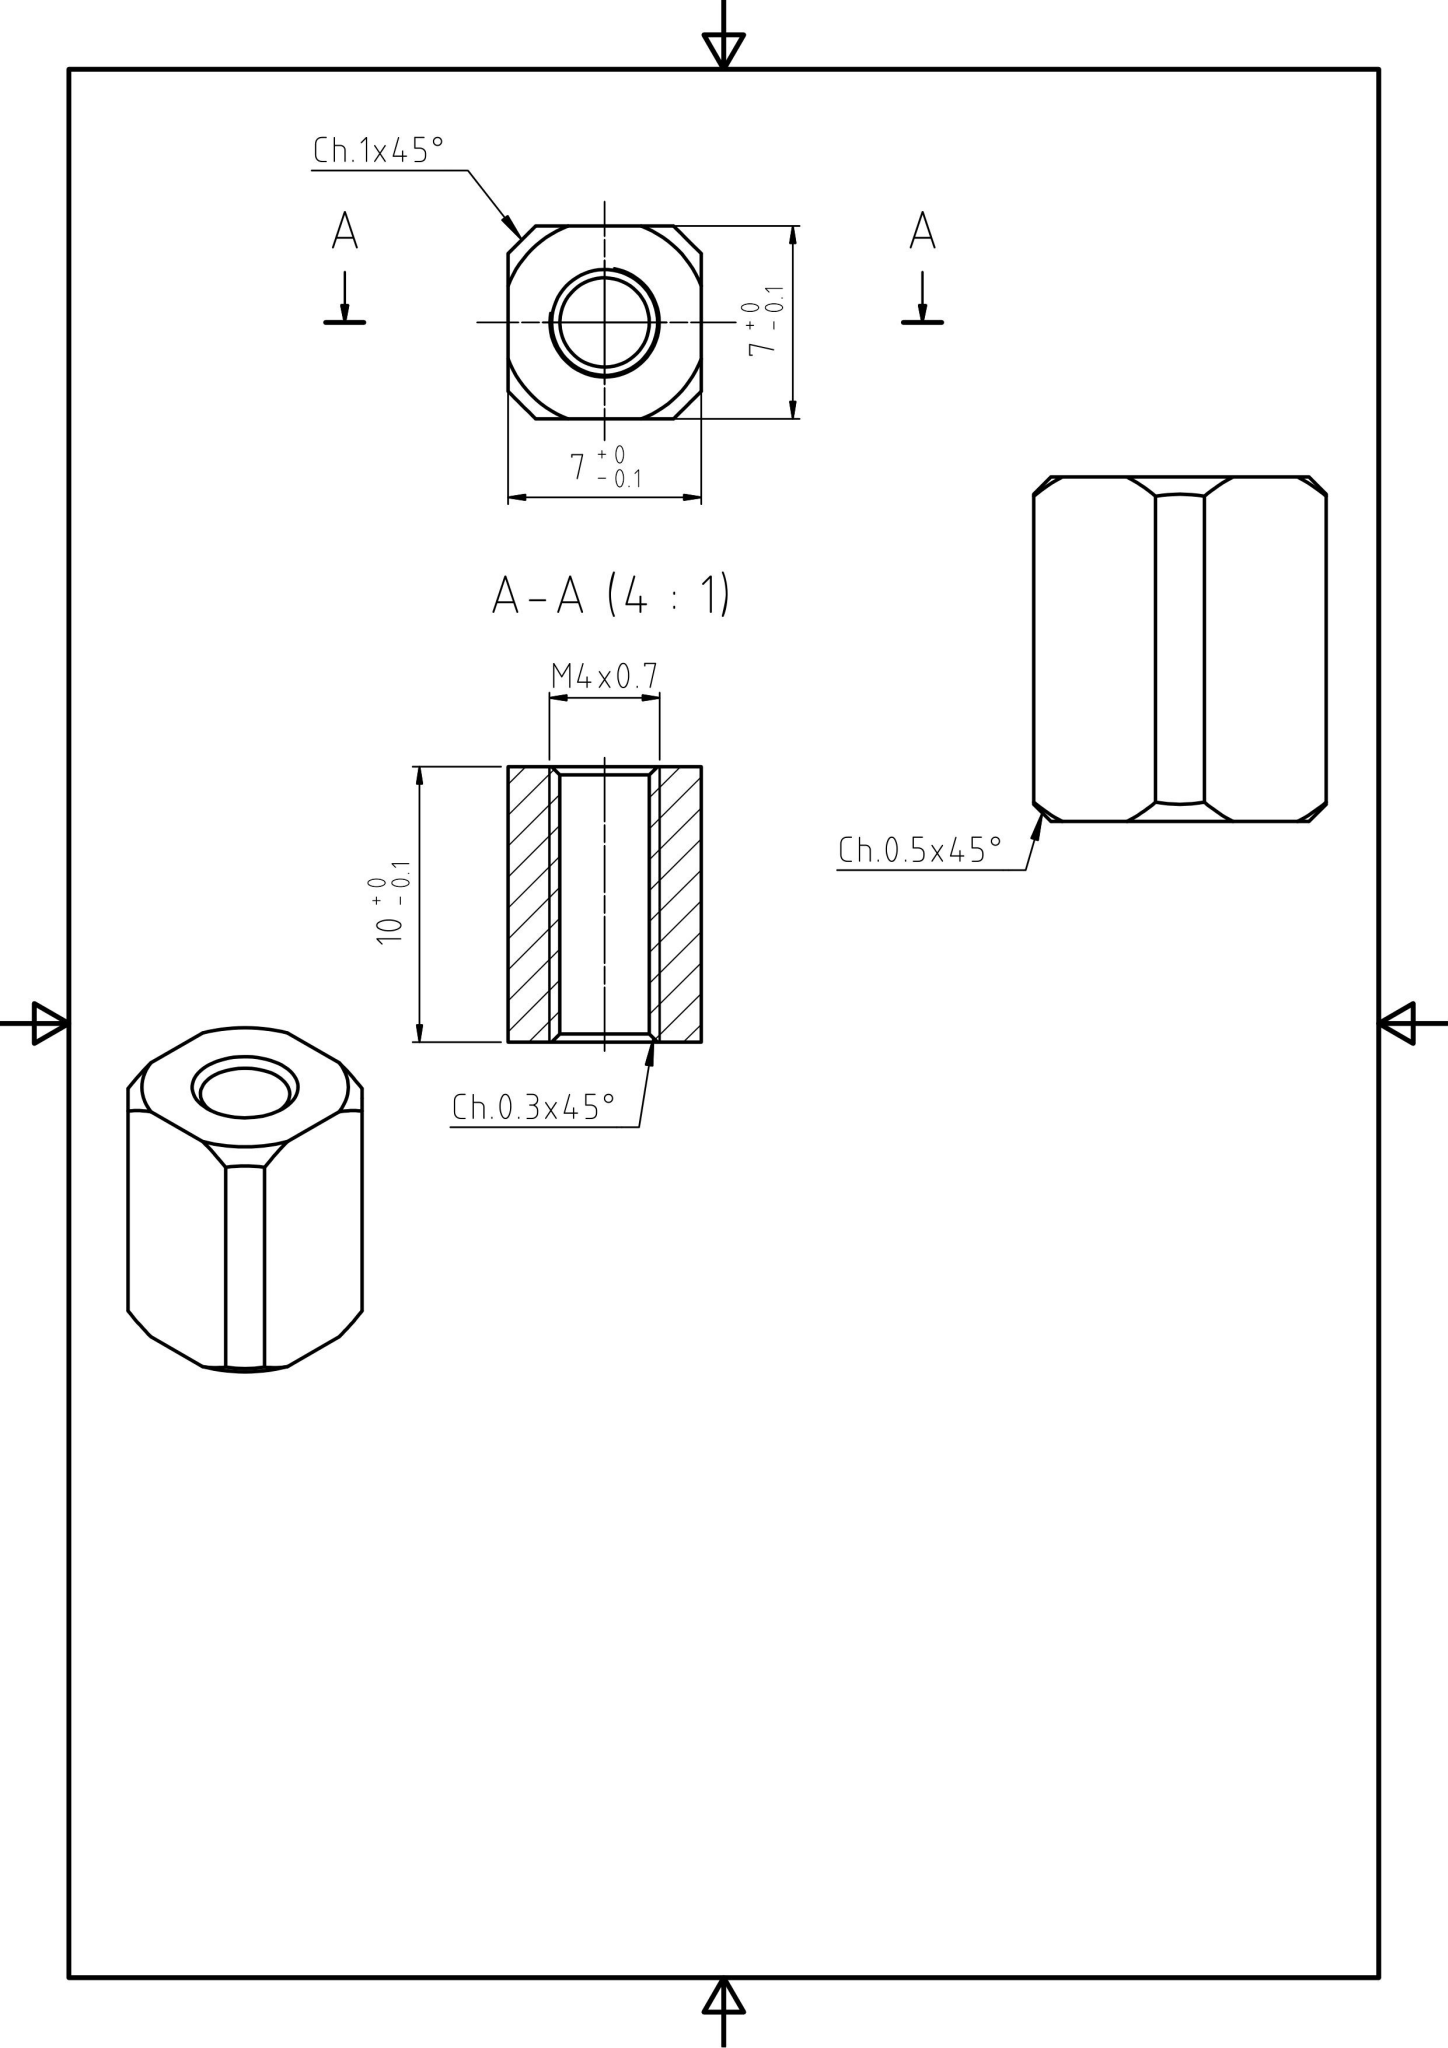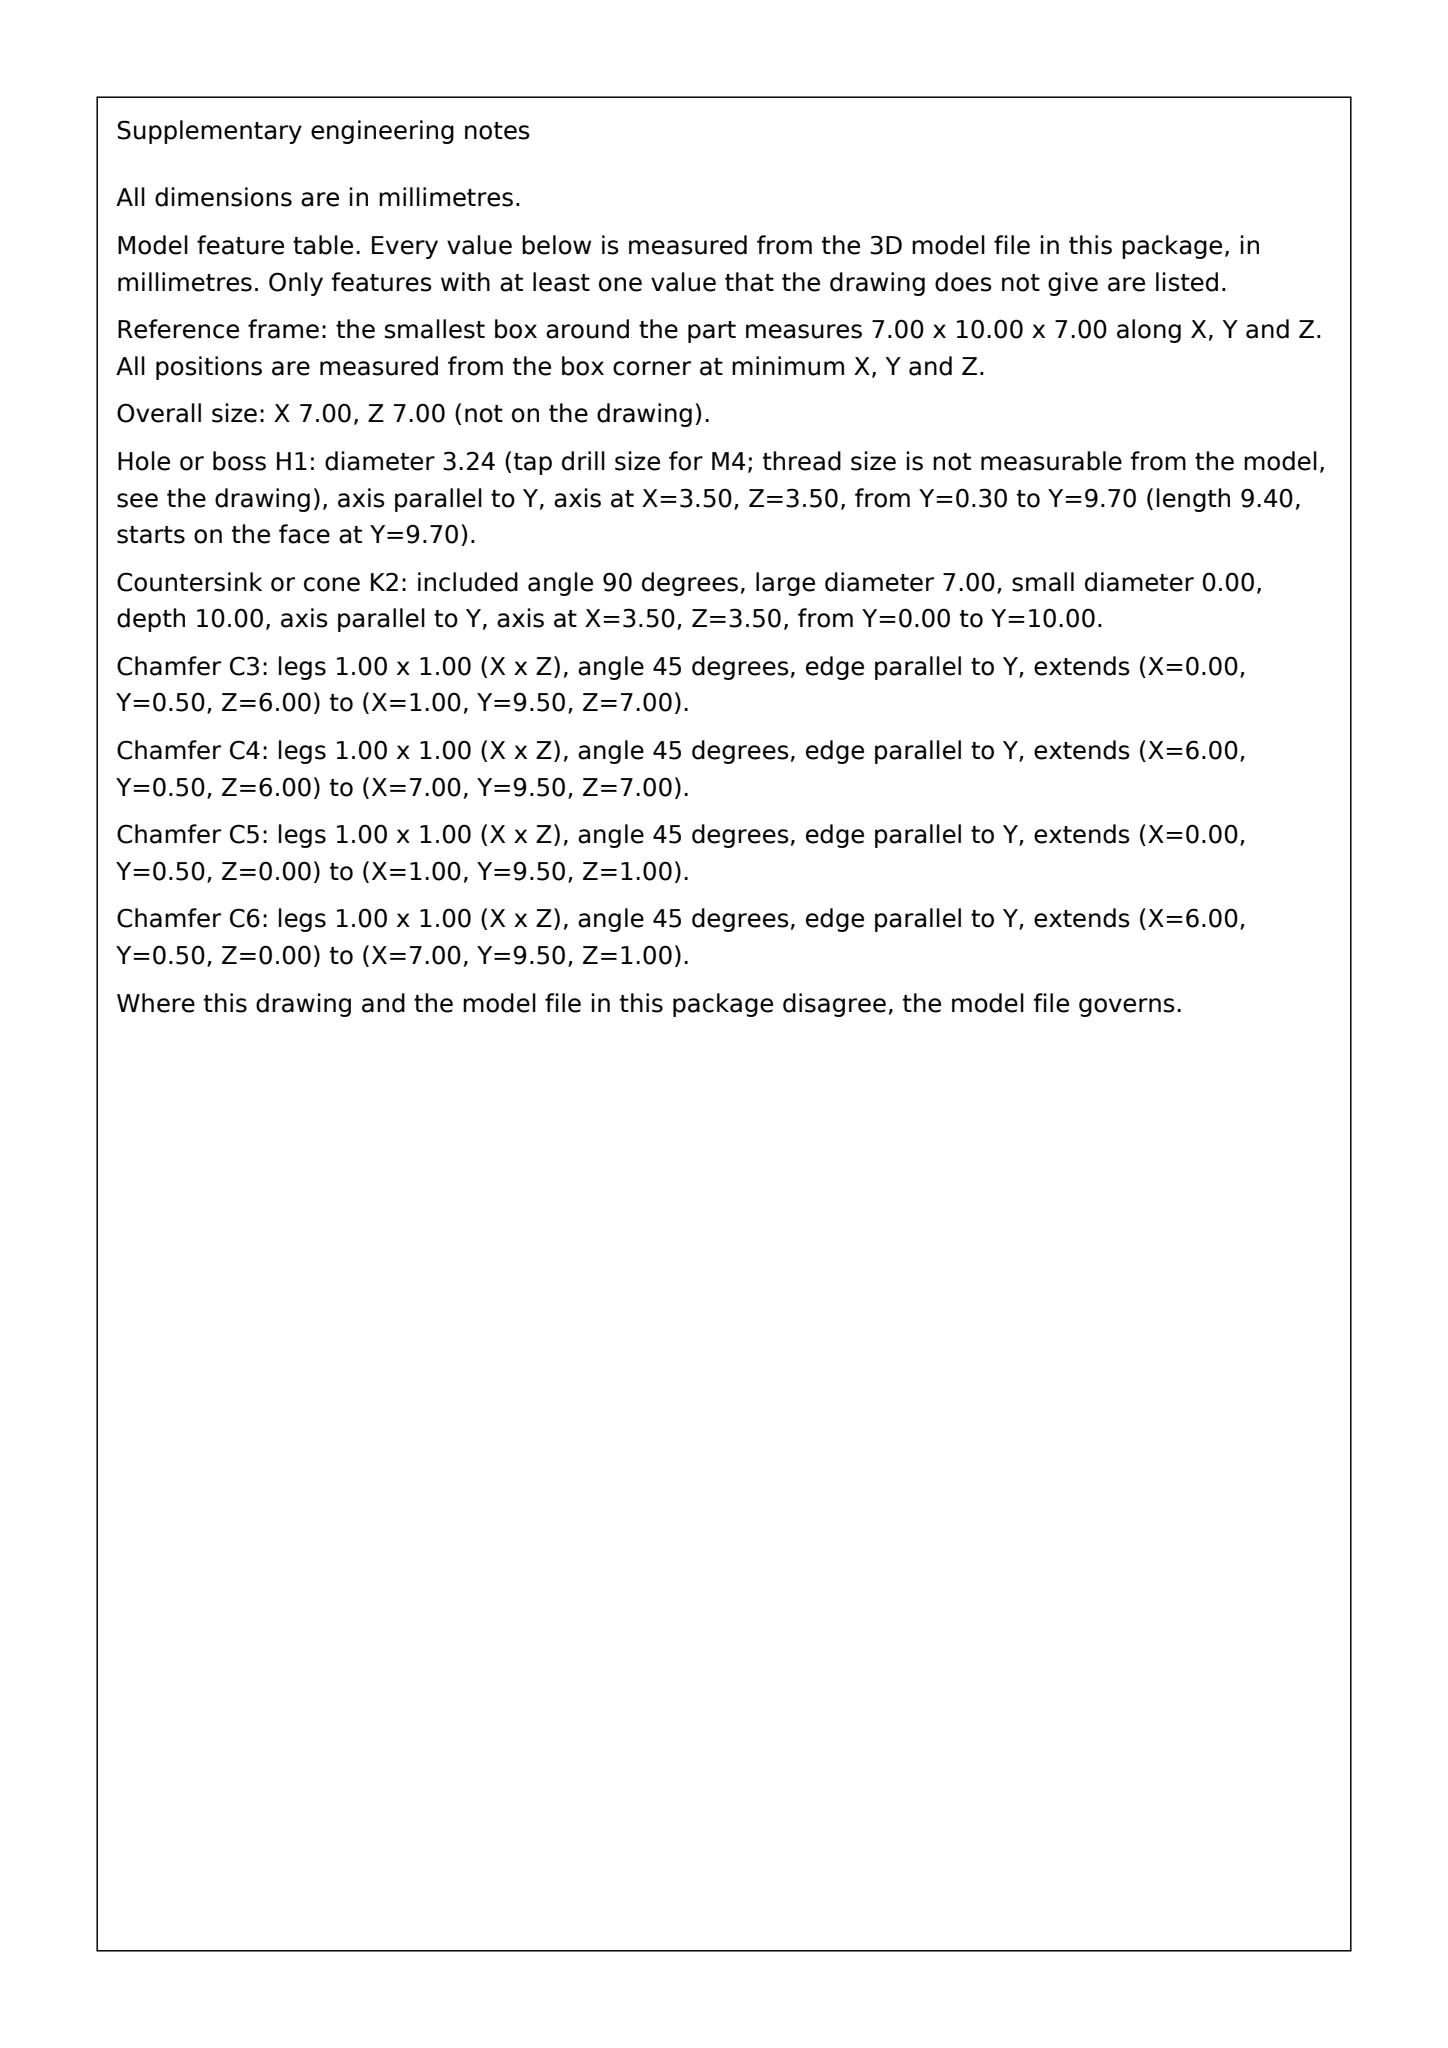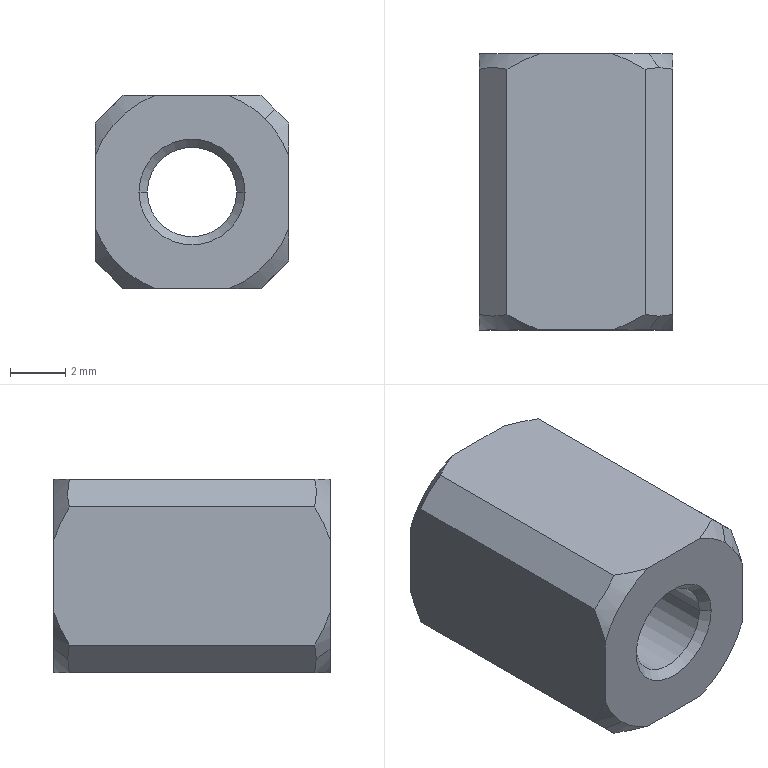Part | SolidWorks | mm | 1 solid | 28 faces | box 7 x 10 x 7 mm | volume 384 mm3 | cone 16 | plane 10 | cylinder 2 | commonest cylinder face diameters 3.242 x2